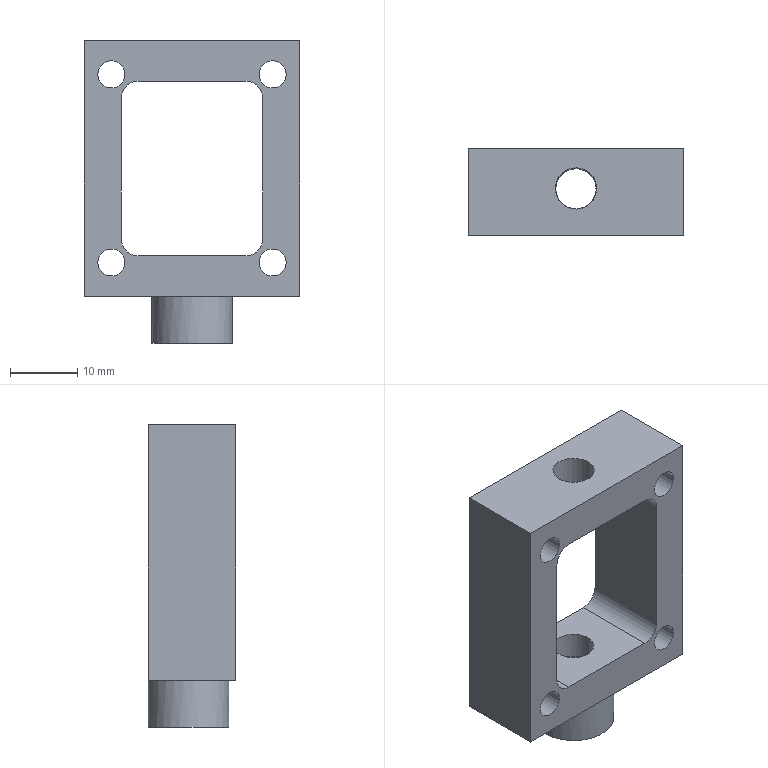Component | NX | OUTER_CONNECTING_BLOCK | 1 solid | 24 faces | volume 8164 mm3 | plane 12 | cylinder 12 | commonest cylinder face diameters 5 x4 4.024 x4 12 x1 6 x1 6.16 x1 8.02 x1